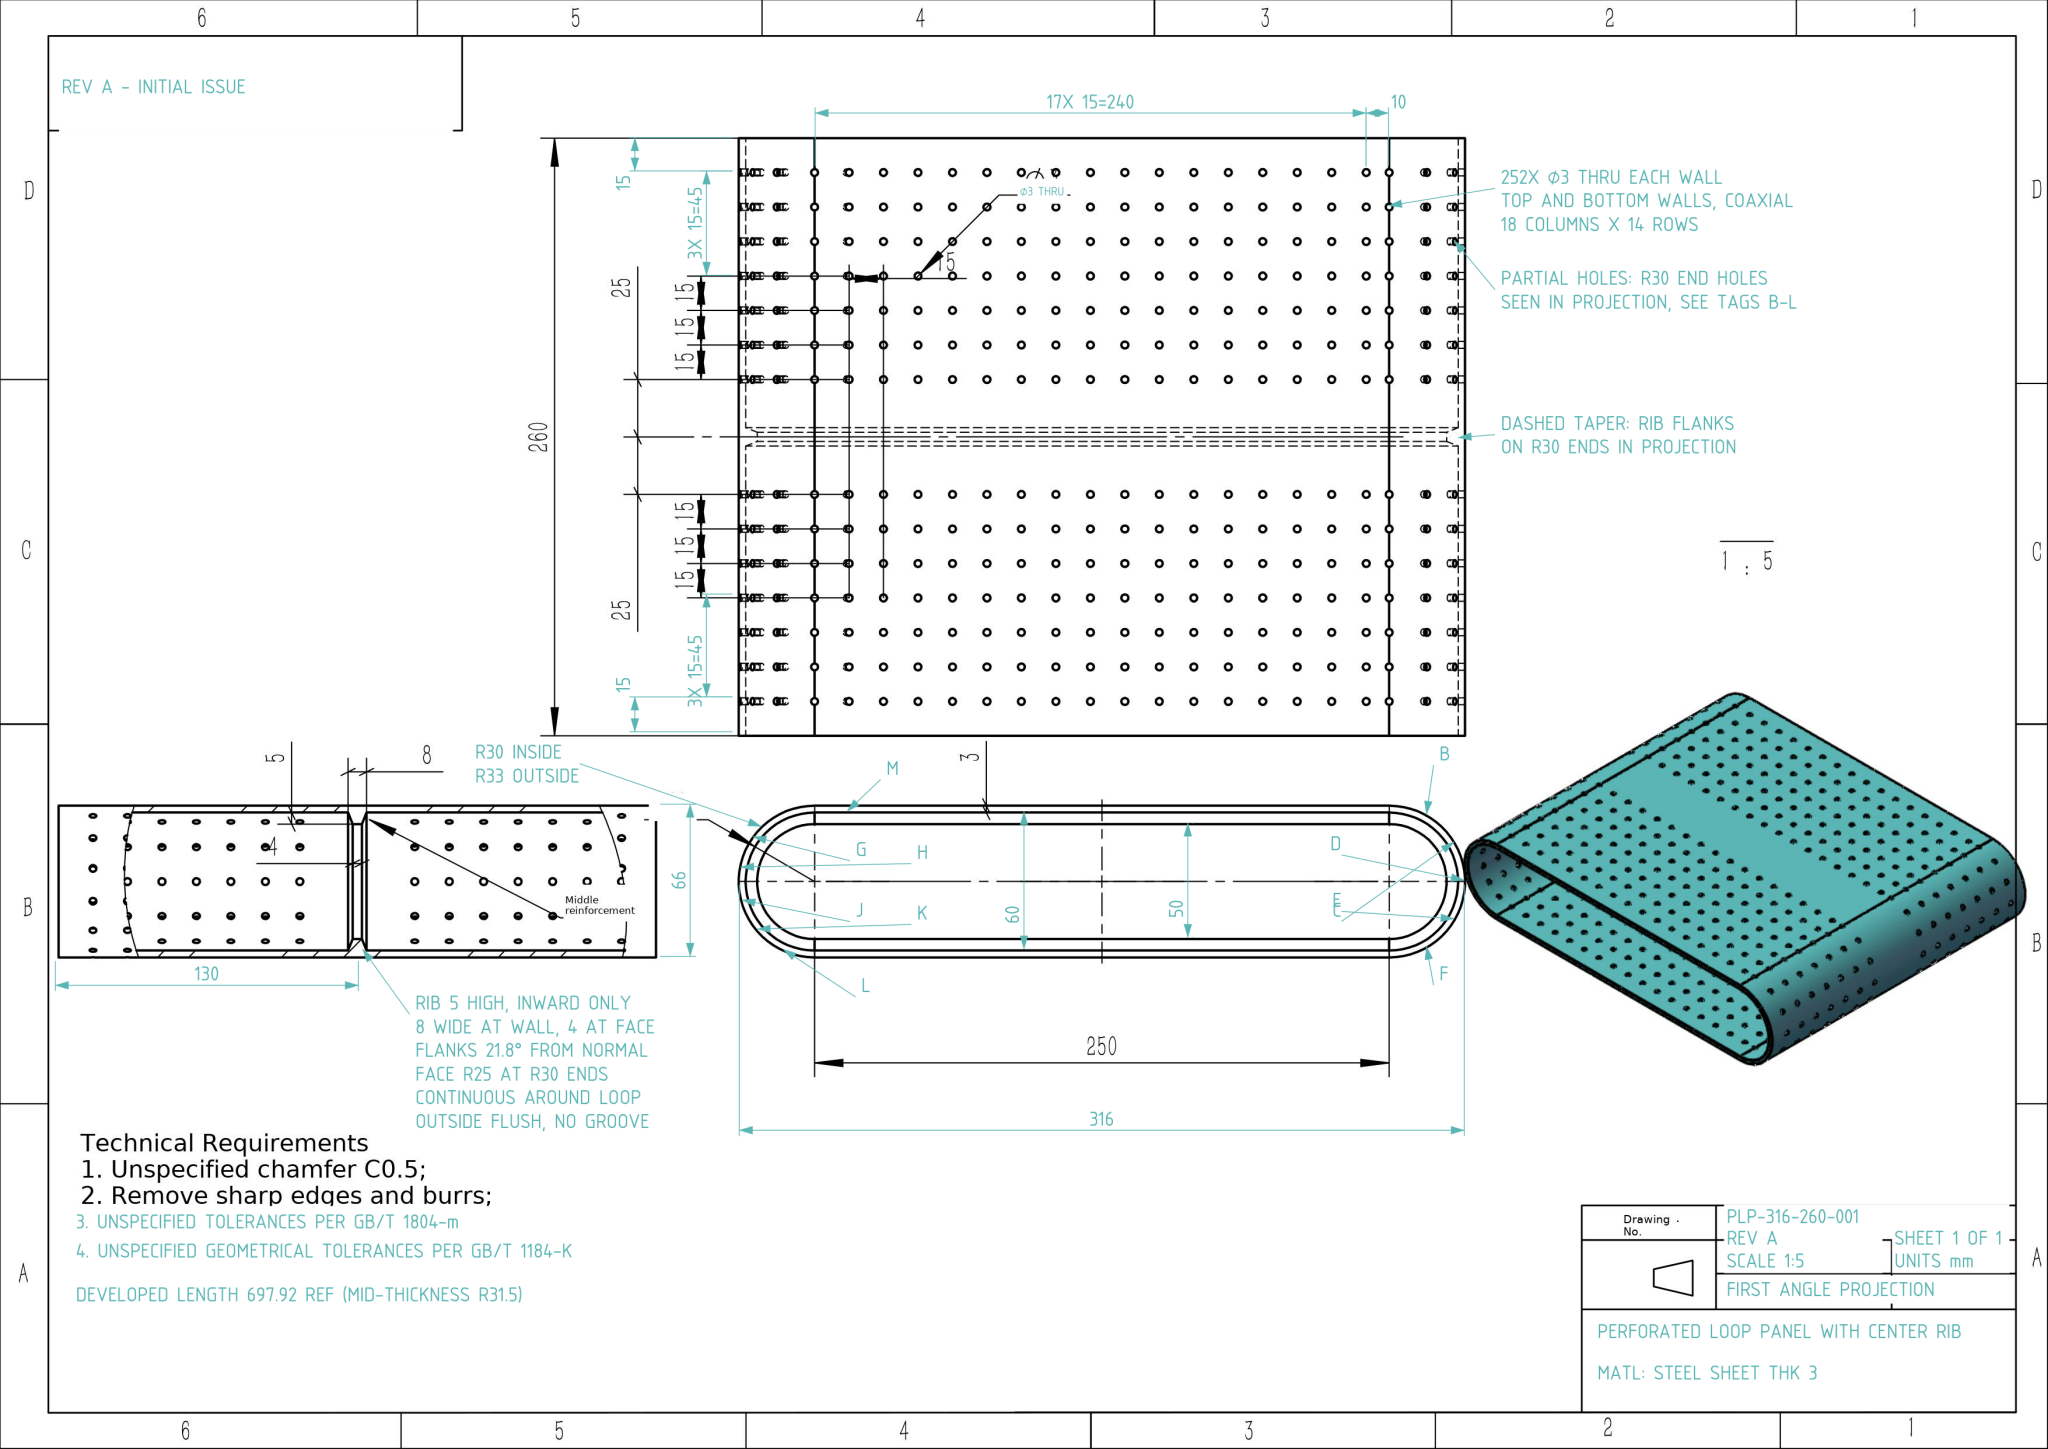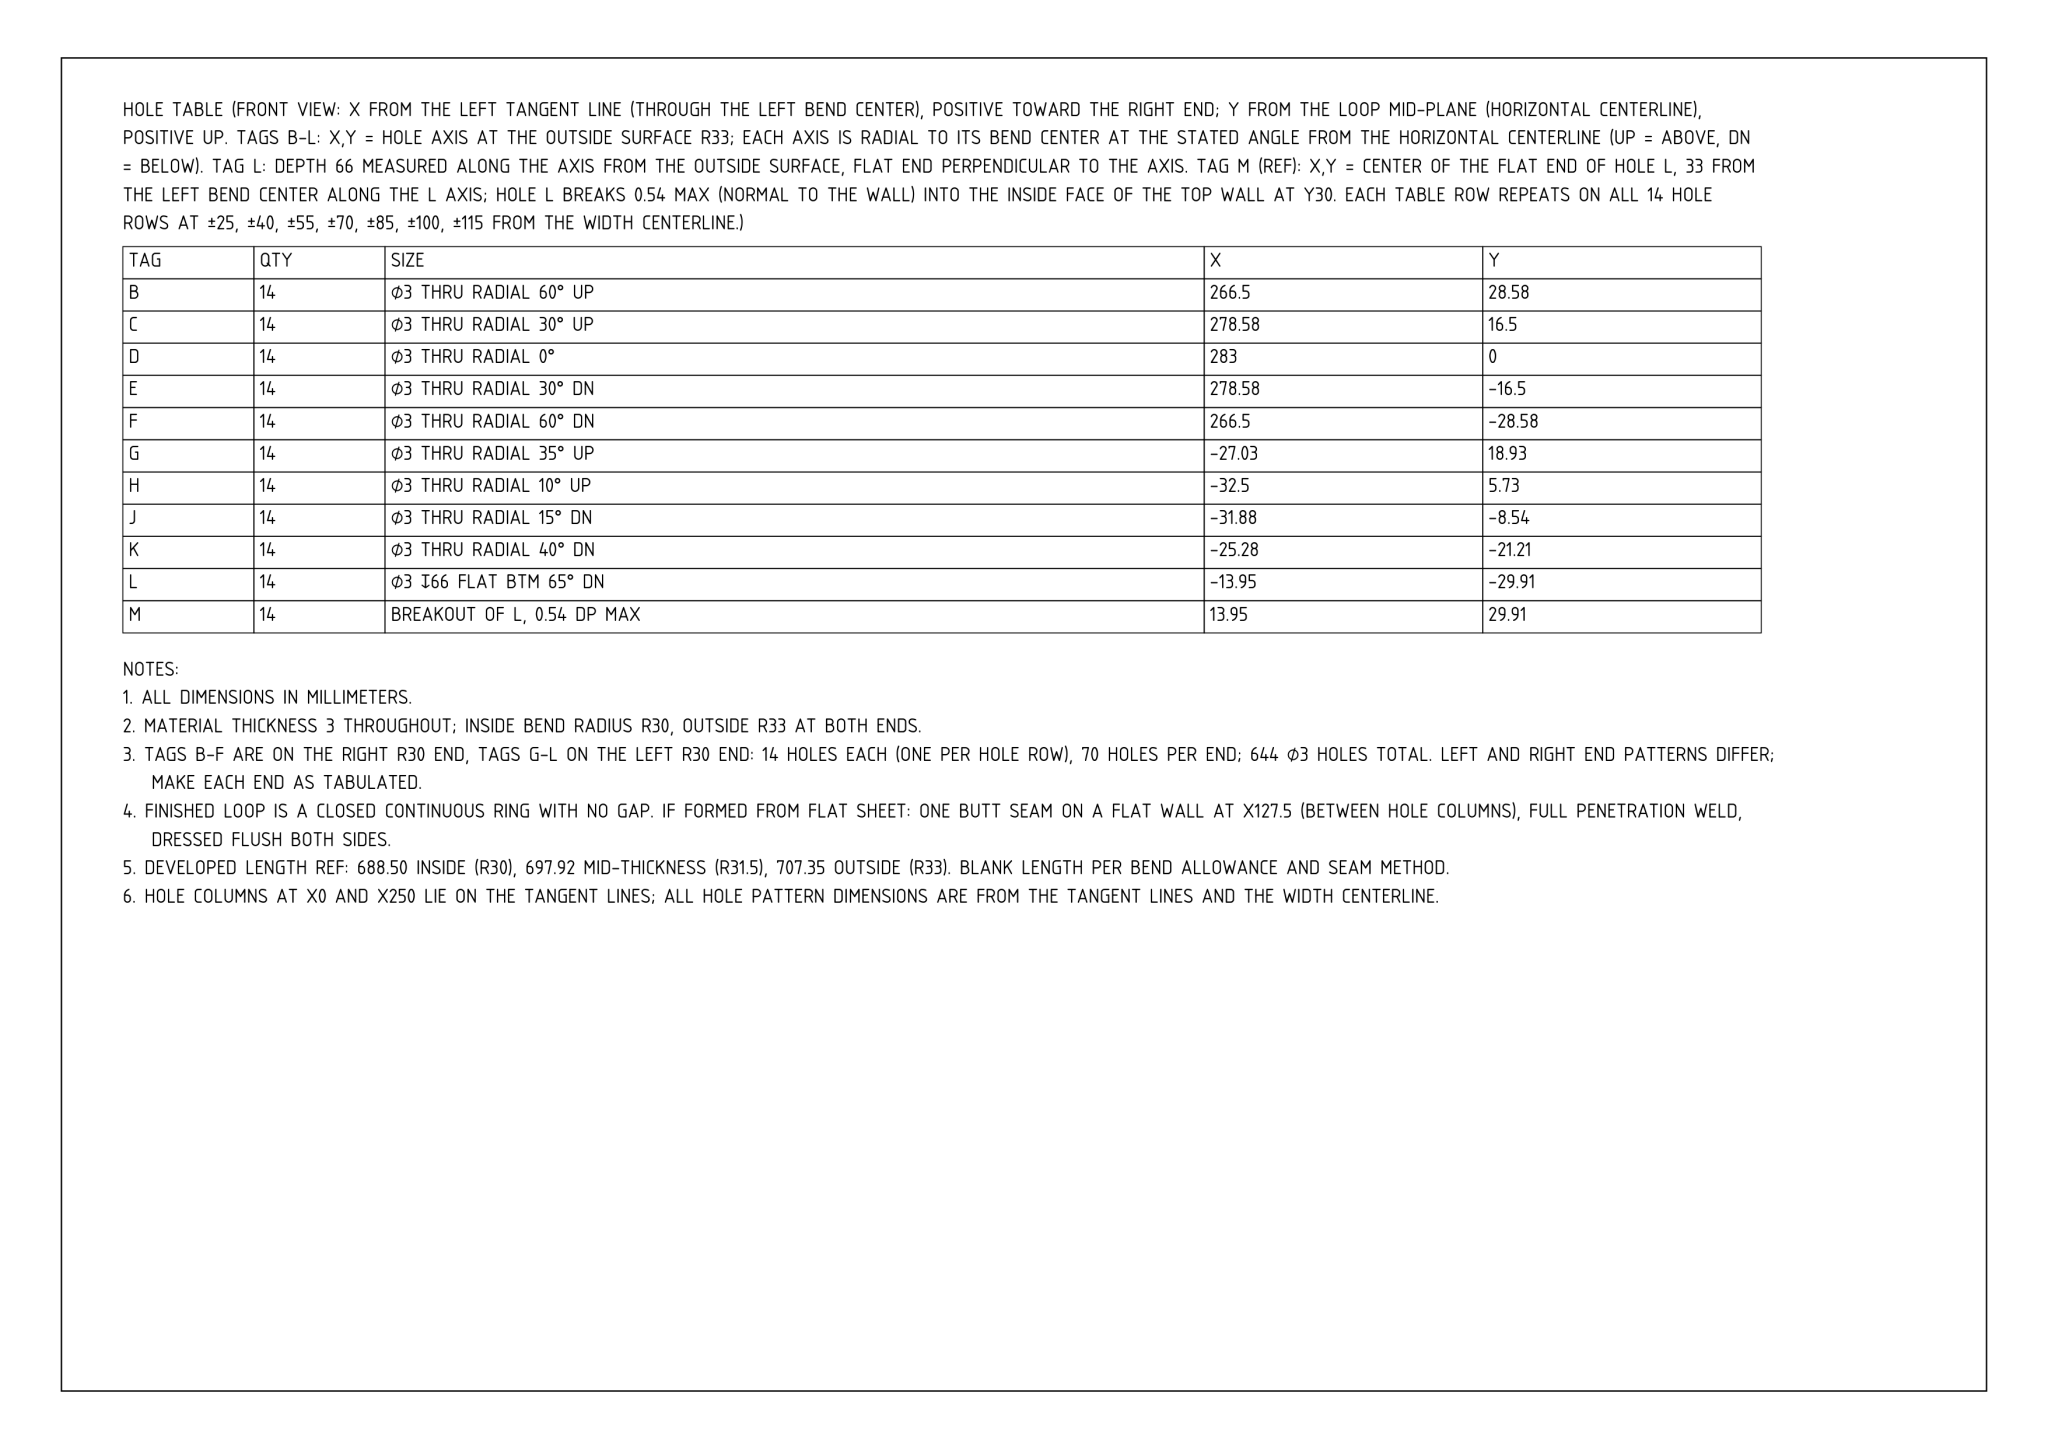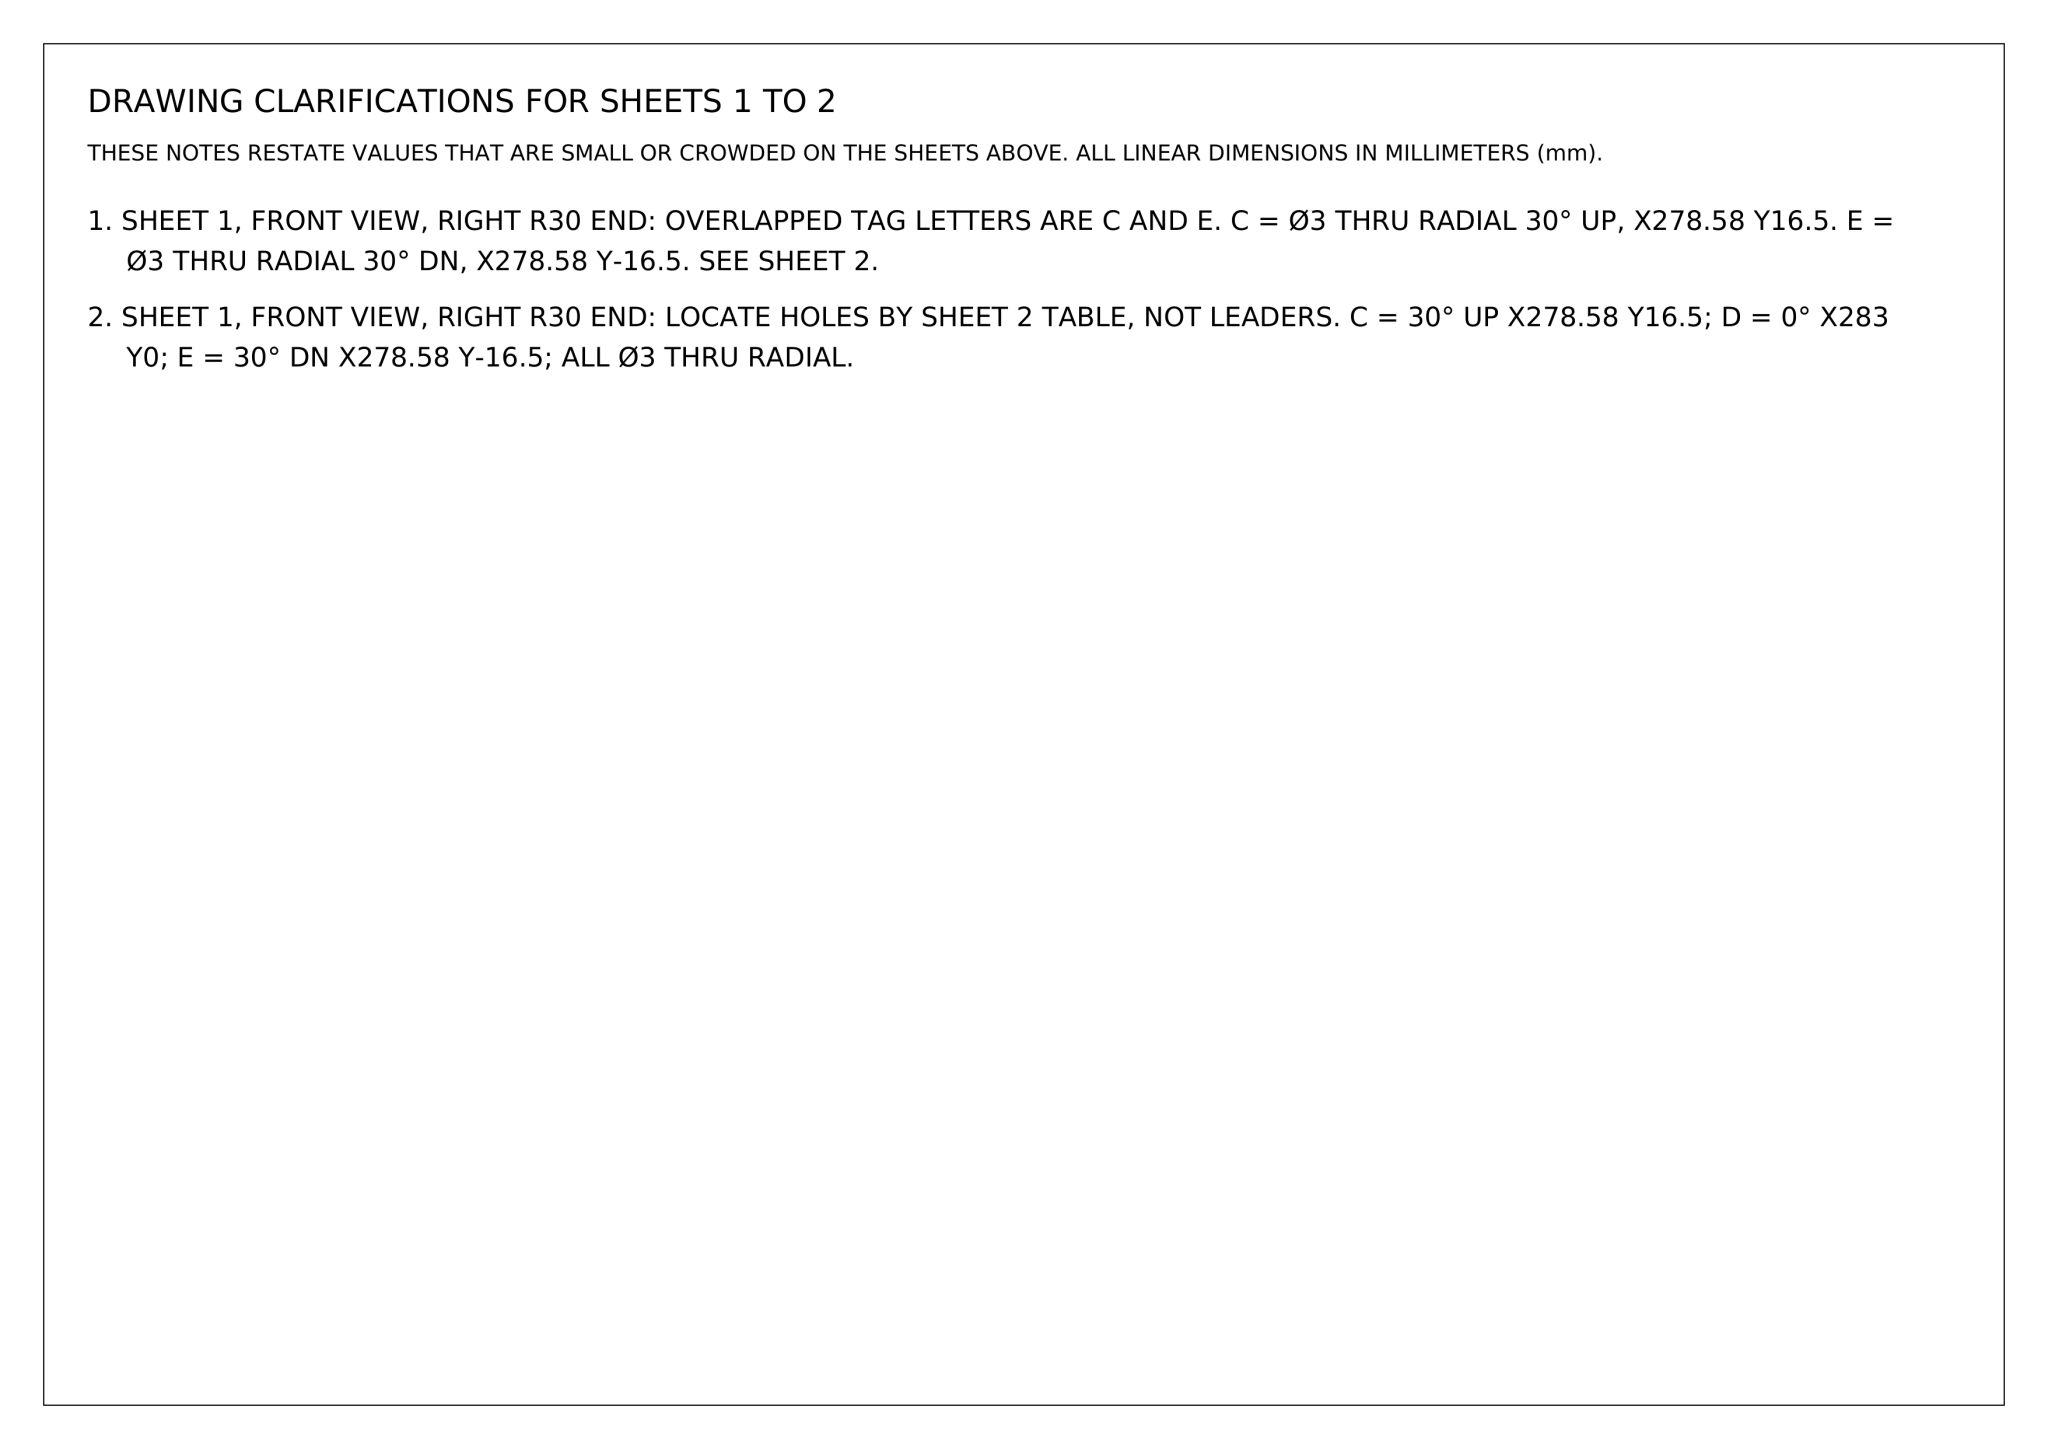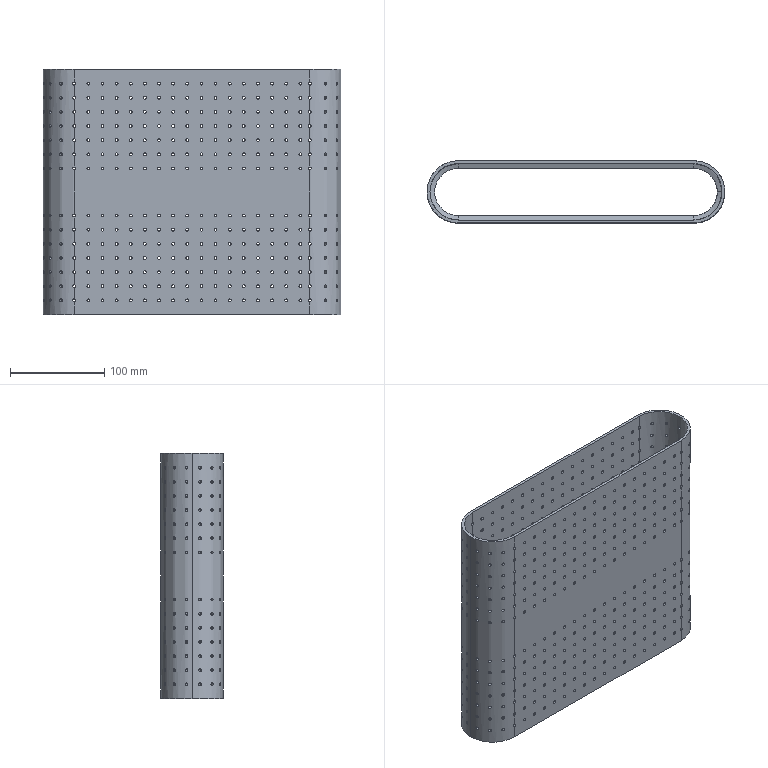Part | NX | mm | 1 solid | 1390 faces | box 316 x 66 x 260 mm | volume 550650 mm3 | cylinder 1356 | plane 28 | cone 6 | commonest cylinder face diameters 3 x1344 60 x6 50 x3 66 x3